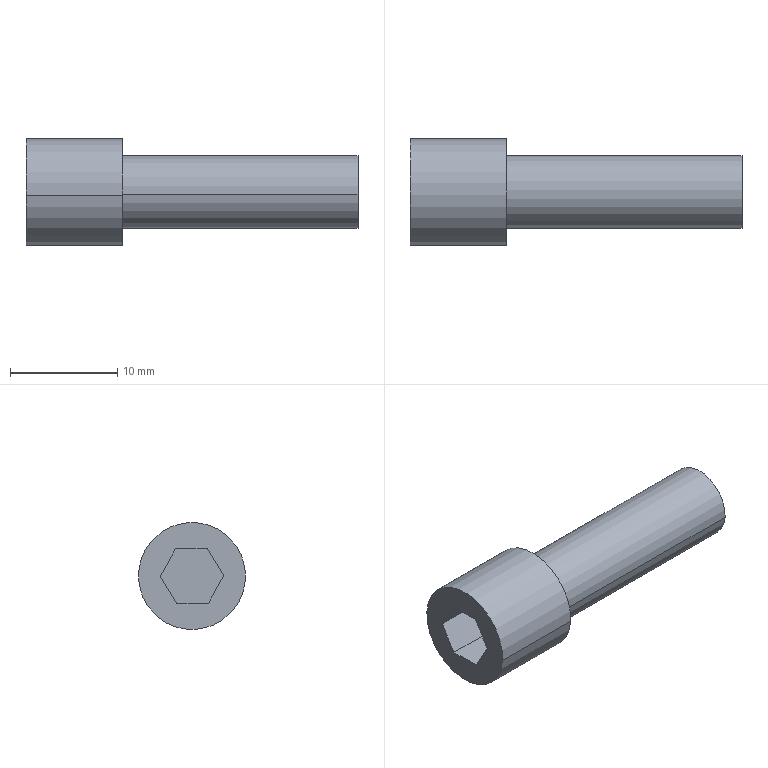Component | SolidWorks | ScrewM8X20-2 | 1 solid | 14 faces | box 31 x 10 x 10 mm | volume 1369 mm3 | plane 10 | cylinder 4 | commonest cylinder face diameters 10 x2 6.8 x2
STEP:
#1=CARTESIAN_POINT('',(-5.315,6.102,-2.114));
#2=VERTEX_POINT('',#1);
#3=CARTESIAN_POINT('',(-5.315,5.709,-2.138));
#4=VERTEX_POINT('',#3);
#5=CARTESIAN_POINT('',(-5.315,5.906,-2.126));
#6=DIRECTION('',(-1.,0.,0.));
#7=DIRECTION('',(0.,0.998,0.06334));
#8=AXIS2_PLACEMENT_3D('',#5,#6,#7);
#9=CIRCLE('',#8,0.1969);
#10=EDGE_CURVE('',#2,#4,#9,.T.);
#11=ORIENTED_EDGE('',*,*,#10,.F.);
#12=CARTESIAN_POINT('',(-4.961,6.102,-2.114));
#13=VERTEX_POINT('',#12);
#14=CARTESIAN_POINT('',(-5.315,6.102,-2.114));
#15=DIRECTION('',(1.,-0.,-0.));
#16=VECTOR('',#15,39.37);
#17=LINE('',#14,#16);
#18=EDGE_CURVE('',#2,#13,#17,.T.);
#19=ORIENTED_EDGE('',*,*,#18,.T.);
#20=CARTESIAN_POINT('',(-4.961,5.709,-2.138));
#21=VERTEX_POINT('',#20);
#22=CARTESIAN_POINT('',(-4.961,5.906,-2.126));
#23=DIRECTION('',(-1.,0.,0.));
#24=DIRECTION('',(0.,0.998,0.06334));
#25=AXIS2_PLACEMENT_3D('',#22,#23,#24);
#26=CIRCLE('',#25,0.1969);
#27=EDGE_CURVE('',#13,#21,#26,.T.);
#28=ORIENTED_EDGE('',*,*,#27,.T.);
#29=CARTESIAN_POINT('',(-5.315,5.709,-2.138));
#30=DIRECTION('',(1.,-0.,-0.));
#31=VECTOR('',#30,39.37);
#32=LINE('',#29,#31);
#33=EDGE_CURVE('',#4,#21,#32,.T.);
#34=ORIENTED_EDGE('',*,*,#33,.F.);
#35=EDGE_LOOP('',(#11,#19,#28,#34));
#36=FACE_OUTER_BOUND('',#35,.T.);
#37=CARTESIAN_POINT('',(-5.315,5.906,-2.126));
#38=DIRECTION('',(1.,-0.,-0.));
#39=DIRECTION('',(0.,-0.998,-0.06334));
#40=AXIS2_PLACEMENT_3D('',#37,#38,#39);
#41=CYLINDRICAL_SURFACE('',#40,0.1969);
#42=ADVANCED_FACE('',(#36),#41,.T.);
#43=CARTESIAN_POINT('',(-4.094,6.039,-2.118));
#44=VERTEX_POINT('',#43);
#45=CARTESIAN_POINT('',(-4.094,5.772,-2.134));
#46=VERTEX_POINT('',#45);
#47=CARTESIAN_POINT('',(-4.094,5.906,-2.126));
#48=DIRECTION('',(-1.,0.,0.));
#49=DIRECTION('',(0.,0.998,0.06334));
#50=AXIS2_PLACEMENT_3D('',#47,#48,#49);
#51=CIRCLE('',#50,0.1339);
#52=EDGE_CURVE('',#44,#46,#51,.T.);
#53=ORIENTED_EDGE('',*,*,#52,.T.);
#54=CARTESIAN_POINT('',(-4.961,5.772,-2.134));
#55=VERTEX_POINT('',#54);
#56=CARTESIAN_POINT('',(-4.094,5.772,-2.134));
#57=DIRECTION('',(-1.,0.,0.));
#58=VECTOR('',#57,39.37);
#59=LINE('',#56,#58);
#60=EDGE_CURVE('',#46,#55,#59,.T.);
#61=ORIENTED_EDGE('',*,*,#60,.T.);
#62=CARTESIAN_POINT('',(-4.961,6.039,-2.118));
#63=VERTEX_POINT('',#62);
#64=CARTESIAN_POINT('',(-4.961,5.906,-2.126));
#65=DIRECTION('',(-1.,0.,0.));
#66=DIRECTION('',(0.,0.998,0.06334));
#67=AXIS2_PLACEMENT_3D('',#64,#65,#66);
#68=CIRCLE('',#67,0.1339);
#69=EDGE_CURVE('',#63,#55,#68,.T.);
#70=ORIENTED_EDGE('',*,*,#69,.F.);
#71=CARTESIAN_POINT('',(-4.094,6.039,-2.118));
#72=DIRECTION('',(-1.,0.,0.));
#73=VECTOR('',#72,39.37);
#74=LINE('',#71,#73);
#75=EDGE_CURVE('',#44,#63,#74,.T.);
#76=ORIENTED_EDGE('',*,*,#75,.F.);
#77=EDGE_LOOP('',(#53,#61,#70,#76));
#78=FACE_OUTER_BOUND('',#77,.T.);
#79=CARTESIAN_POINT('',(-4.094,5.906,-2.126));
#80=DIRECTION('',(-1.,0.,0.));
#81=DIRECTION('',(0.,0.998,0.06334));
#82=AXIS2_PLACEMENT_3D('',#79,#80,#81);
#83=CYLINDRICAL_SURFACE('',#82,0.1339);
#84=ADVANCED_FACE('',(#78),#83,.T.);
#85=ORIENTED_EDGE('',*,*,#60,.F.);
#86=CARTESIAN_POINT('',(-4.094,5.906,-2.126));
#87=DIRECTION('',(-1.,0.,0.));
#88=DIRECTION('',(0.,0.998,0.06334));
#89=AXIS2_PLACEMENT_3D('',#86,#87,#88);
#90=CIRCLE('',#89,0.1339);
#91=EDGE_CURVE('',#46,#44,#90,.T.);
#92=ORIENTED_EDGE('',*,*,#91,.T.);
#93=ORIENTED_EDGE('',*,*,#75,.T.);
#94=CARTESIAN_POINT('',(-4.961,5.906,-2.126));
#95=DIRECTION('',(-1.,0.,0.));
#96=DIRECTION('',(0.,0.998,0.06334));
#97=AXIS2_PLACEMENT_3D('',#94,#95,#96);
#98=CIRCLE('',#97,0.1339);
#99=EDGE_CURVE('',#55,#63,#98,.T.);
#100=ORIENTED_EDGE('',*,*,#99,.F.);
#101=EDGE_LOOP('',(#85,#92,#93,#100));
#102=FACE_OUTER_BOUND('',#101,.T.);
#103=CARTESIAN_POINT('',(-4.094,5.906,-2.126));
#104=DIRECTION('',(-1.,0.,0.));
#105=DIRECTION('',(0.,0.998,0.06334));
#106=AXIS2_PLACEMENT_3D('',#103,#104,#105);
#107=CYLINDRICAL_SURFACE('',#106,0.1339);
#108=ADVANCED_FACE('',(#102),#107,.T.);
#109=ORIENTED_EDGE('',*,*,#52,.F.);
#110=ORIENTED_EDGE('',*,*,#91,.F.);
#111=EDGE_LOOP('',(#109,#110));
#112=FACE_OUTER_BOUND('',#111,.T.);
#113=CARTESIAN_POINT('',(-4.094,5.906,-2.126));
#114=DIRECTION('',(-1.,0.,0.));
#115=DIRECTION('',(0.,0.998,0.06334));
#116=AXIS2_PLACEMENT_3D('',#113,#114,#115);
#117=PLANE('',#116);
#118=ADVANCED_FACE('',(#112),#117,.F.);
#119=ORIENTED_EDGE('',*,*,#18,.F.);
#120=CARTESIAN_POINT('',(-5.315,5.906,-2.126));
#121=DIRECTION('',(-1.,0.,0.));
#122=DIRECTION('',(0.,0.998,0.06334));
#123=AXIS2_PLACEMENT_3D('',#120,#121,#122);
#124=CIRCLE('',#123,0.1969);
#125=EDGE_CURVE('',#4,#2,#124,.T.);
#126=ORIENTED_EDGE('',*,*,#125,.F.);
#127=ORIENTED_EDGE('',*,*,#33,.T.);
#128=CARTESIAN_POINT('',(-4.961,5.906,-2.126));
#129=DIRECTION('',(-1.,0.,0.));
#130=DIRECTION('',(0.,0.998,0.06334));
#131=AXIS2_PLACEMENT_3D('',#128,#129,#130);
#132=CIRCLE('',#131,0.1969);
#133=EDGE_CURVE('',#21,#13,#132,.T.);
#134=ORIENTED_EDGE('',*,*,#133,.T.);
#135=EDGE_LOOP('',(#119,#126,#127,#134));
#136=FACE_OUTER_BOUND('',#135,.T.);
#137=CARTESIAN_POINT('',(-5.315,5.906,-2.126));
#138=DIRECTION('',(1.,-0.,-0.));
#139=DIRECTION('',(0.,-0.998,-0.06334));
#140=AXIS2_PLACEMENT_3D('',#137,#138,#139);
#141=CYLINDRICAL_SURFACE('',#140,0.1969);
#142=ADVANCED_FACE('',(#136),#141,.T.);
#143=CARTESIAN_POINT('',(-5.315,6.022,-2.129));
#144=VERTEX_POINT('',#143);
#145=CARTESIAN_POINT('',(-5.315,5.962,-2.228));
#146=VERTEX_POINT('',#145);
#147=CARTESIAN_POINT('',(-5.315,6.022,-2.129));
#148=DIRECTION('',(-0.,-0.5195,-0.8544));
#149=VECTOR('',#148,39.37);
#150=LINE('',#147,#149);
#151=EDGE_CURVE('',#144,#146,#150,.T.);
#152=ORIENTED_EDGE('',*,*,#151,.F.);
#153=CARTESIAN_POINT('',(-5.315,5.966,-2.026));
#154=VERTEX_POINT('',#153);
#155=CARTESIAN_POINT('',(-5.315,5.966,-2.026));
#156=DIRECTION('',(-0.,0.4802,-0.8772));
#157=VECTOR('',#156,39.37);
#158=LINE('',#155,#157);
#159=EDGE_CURVE('',#154,#144,#158,.T.);
#160=ORIENTED_EDGE('',*,*,#159,.F.);
#161=CARTESIAN_POINT('',(-5.315,5.849,-2.024));
#162=VERTEX_POINT('',#161);
#163=CARTESIAN_POINT('',(-5.315,5.849,-2.024));
#164=DIRECTION('',(0.,0.9997,-0.02271));
#165=VECTOR('',#164,39.37);
#166=LINE('',#163,#165);
#167=EDGE_CURVE('',#162,#154,#166,.T.);
#168=ORIENTED_EDGE('',*,*,#167,.F.);
#169=CARTESIAN_POINT('',(-5.315,5.789,-2.123));
#170=VERTEX_POINT('',#169);
#171=CARTESIAN_POINT('',(-5.315,5.789,-2.123));
#172=DIRECTION('',(0.,0.5195,0.8544));
#173=VECTOR('',#172,39.37);
#174=LINE('',#171,#173);
#175=EDGE_CURVE('',#170,#162,#174,.T.);
#176=ORIENTED_EDGE('',*,*,#175,.F.);
#177=CARTESIAN_POINT('',(-5.315,5.845,-2.226));
#178=VERTEX_POINT('',#177);
#179=CARTESIAN_POINT('',(-5.315,5.845,-2.226));
#180=DIRECTION('',(0.,-0.4802,0.8772));
#181=VECTOR('',#180,39.37);
#182=LINE('',#179,#181);
#183=EDGE_CURVE('',#178,#170,#182,.T.);
#184=ORIENTED_EDGE('',*,*,#183,.F.);
#185=CARTESIAN_POINT('',(-5.315,5.962,-2.228));
#186=DIRECTION('',(-0.,-0.9997,0.02271));
#187=VECTOR('',#186,39.37);
#188=LINE('',#185,#187);
#189=EDGE_CURVE('',#146,#178,#188,.T.);
#190=ORIENTED_EDGE('',*,*,#189,.F.);
#191=EDGE_LOOP('',(#152,#160,#168,#176,#184,#190));
#192=FACE_BOUND('',#191,.T.);
#193=ORIENTED_EDGE('',*,*,#125,.T.);
#194=ORIENTED_EDGE('',*,*,#10,.T.);
#195=EDGE_LOOP('',(#193,#194));
#196=FACE_OUTER_BOUND('',#195,.T.);
#197=CARTESIAN_POINT('',(-5.315,5.906,-2.126));
#198=DIRECTION('',(-1.,0.,0.));
#199=DIRECTION('',(0.,0.998,0.06334));
#200=AXIS2_PLACEMENT_3D('',#197,#198,#199);
#201=PLANE('',#200);
#202=ADVANCED_FACE('',(#192,#196),#201,.T.);
#203=ORIENTED_EDGE('',*,*,#69,.T.);
#204=ORIENTED_EDGE('',*,*,#99,.T.);
#205=EDGE_LOOP('',(#203,#204));
#206=FACE_BOUND('',#205,.T.);
#207=ORIENTED_EDGE('',*,*,#133,.F.);
#208=ORIENTED_EDGE('',*,*,#27,.F.);
#209=EDGE_LOOP('',(#207,#208));
#210=FACE_OUTER_BOUND('',#209,.T.);
#211=CARTESIAN_POINT('',(-4.961,5.906,-2.126));
#212=DIRECTION('',(-1.,0.,0.));
#213=DIRECTION('',(0.,0.998,0.06334));
#214=AXIS2_PLACEMENT_3D('',#211,#212,#213);
#215=PLANE('',#214);
#216=ADVANCED_FACE('',(#206,#210),#215,.F.);
#217=ORIENTED_EDGE('',*,*,#151,.T.);
#218=CARTESIAN_POINT('',(-5.079,5.962,-2.228));
#219=VERTEX_POINT('',#218);
#220=CARTESIAN_POINT('',(-5.079,5.962,-2.228));
#221=DIRECTION('',(-1.,0.,0.));
#222=VECTOR('',#221,39.37);
#223=LINE('',#220,#222);
#224=EDGE_CURVE('',#219,#146,#223,.T.);
#225=ORIENTED_EDGE('',*,*,#224,.F.);
#226=CARTESIAN_POINT('',(-5.079,6.022,-2.129));
#227=VERTEX_POINT('',#226);
#228=CARTESIAN_POINT('',(-5.079,6.022,-2.129));
#229=DIRECTION('',(-0.,-0.5195,-0.8544));
#230=VECTOR('',#229,39.37);
#231=LINE('',#228,#230);
#232=EDGE_CURVE('',#227,#219,#231,.T.);
#233=ORIENTED_EDGE('',*,*,#232,.F.);
#234=CARTESIAN_POINT('',(-5.079,6.022,-2.129));
#235=DIRECTION('',(-1.,0.,0.));
#236=VECTOR('',#235,39.37);
#237=LINE('',#234,#236);
#238=EDGE_CURVE('',#227,#144,#237,.T.);
#239=ORIENTED_EDGE('',*,*,#238,.T.);
#240=EDGE_LOOP('',(#217,#225,#233,#239));
#241=FACE_OUTER_BOUND('',#240,.T.);
#242=CARTESIAN_POINT('',(-5.079,6.022,-2.129));
#243=DIRECTION('',(0.,0.8544,-0.5195));
#244=DIRECTION('',(-0.,-0.5195,-0.8544));
#245=AXIS2_PLACEMENT_3D('',#242,#243,#244);
#246=PLANE('',#245);
#247=ADVANCED_FACE('',(#241),#246,.F.);
#248=ORIENTED_EDGE('',*,*,#159,.T.);
#249=ORIENTED_EDGE('',*,*,#238,.F.);
#250=CARTESIAN_POINT('',(-5.079,5.966,-2.026));
#251=VERTEX_POINT('',#250);
#252=CARTESIAN_POINT('',(-5.079,5.966,-2.026));
#253=DIRECTION('',(-0.,0.4802,-0.8772));
#254=VECTOR('',#253,39.37);
#255=LINE('',#252,#254);
#256=EDGE_CURVE('',#251,#227,#255,.T.);
#257=ORIENTED_EDGE('',*,*,#256,.F.);
#258=CARTESIAN_POINT('',(-5.079,5.966,-2.026));
#259=DIRECTION('',(-1.,0.,0.));
#260=VECTOR('',#259,39.37);
#261=LINE('',#258,#260);
#262=EDGE_CURVE('',#251,#154,#261,.T.);
#263=ORIENTED_EDGE('',*,*,#262,.T.);
#264=EDGE_LOOP('',(#248,#249,#257,#263));
#265=FACE_OUTER_BOUND('',#264,.T.);
#266=CARTESIAN_POINT('',(-5.079,5.966,-2.026));
#267=DIRECTION('',(0.,0.8772,0.4802));
#268=DIRECTION('',(-0.,0.4802,-0.8772));
#269=AXIS2_PLACEMENT_3D('',#266,#267,#268);
#270=PLANE('',#269);
#271=ADVANCED_FACE('',(#265),#270,.F.);
#272=ORIENTED_EDGE('',*,*,#167,.T.);
#273=ORIENTED_EDGE('',*,*,#262,.F.);
#274=CARTESIAN_POINT('',(-5.079,5.849,-2.024));
#275=VERTEX_POINT('',#274);
#276=CARTESIAN_POINT('',(-5.079,5.849,-2.024));
#277=DIRECTION('',(0.,0.9997,-0.02271));
#278=VECTOR('',#277,39.37);
#279=LINE('',#276,#278);
#280=EDGE_CURVE('',#275,#251,#279,.T.);
#281=ORIENTED_EDGE('',*,*,#280,.F.);
#282=CARTESIAN_POINT('',(-5.079,5.849,-2.024));
#283=DIRECTION('',(-1.,0.,0.));
#284=VECTOR('',#283,39.37);
#285=LINE('',#282,#284);
#286=EDGE_CURVE('',#275,#162,#285,.T.);
#287=ORIENTED_EDGE('',*,*,#286,.T.);
#288=EDGE_LOOP('',(#272,#273,#281,#287));
#289=FACE_OUTER_BOUND('',#288,.T.);
#290=CARTESIAN_POINT('',(-5.079,5.849,-2.024));
#291=DIRECTION('',(0.,0.02271,0.9997));
#292=DIRECTION('',(0.,0.9997,-0.02271));
#293=AXIS2_PLACEMENT_3D('',#290,#291,#292);
#294=PLANE('',#293);
#295=ADVANCED_FACE('',(#289),#294,.F.);
#296=ORIENTED_EDGE('',*,*,#175,.T.);
#297=ORIENTED_EDGE('',*,*,#286,.F.);
#298=CARTESIAN_POINT('',(-5.079,5.789,-2.123));
#299=VERTEX_POINT('',#298);
#300=CARTESIAN_POINT('',(-5.079,5.789,-2.123));
#301=DIRECTION('',(0.,0.5195,0.8544));
#302=VECTOR('',#301,39.37);
#303=LINE('',#300,#302);
#304=EDGE_CURVE('',#299,#275,#303,.T.);
#305=ORIENTED_EDGE('',*,*,#304,.F.);
#306=CARTESIAN_POINT('',(-5.079,5.789,-2.123));
#307=DIRECTION('',(-1.,0.,0.));
#308=VECTOR('',#307,39.37);
#309=LINE('',#306,#308);
#310=EDGE_CURVE('',#299,#170,#309,.T.);
#311=ORIENTED_EDGE('',*,*,#310,.T.);
#312=EDGE_LOOP('',(#296,#297,#305,#311));
#313=FACE_OUTER_BOUND('',#312,.T.);
#314=CARTESIAN_POINT('',(-5.079,5.789,-2.123));
#315=DIRECTION('',(-0.,-0.8544,0.5195));
#316=DIRECTION('',(0.,0.5195,0.8544));
#317=AXIS2_PLACEMENT_3D('',#314,#315,#316);
#318=PLANE('',#317);
#319=ADVANCED_FACE('',(#313),#318,.F.);
#320=ORIENTED_EDGE('',*,*,#183,.T.);
#321=ORIENTED_EDGE('',*,*,#310,.F.);
#322=CARTESIAN_POINT('',(-5.079,5.845,-2.226));
#323=VERTEX_POINT('',#322);
#324=CARTESIAN_POINT('',(-5.079,5.845,-2.226));
#325=DIRECTION('',(0.,-0.4802,0.8772));
#326=VECTOR('',#325,39.37);
#327=LINE('',#324,#326);
#328=EDGE_CURVE('',#323,#299,#327,.T.);
#329=ORIENTED_EDGE('',*,*,#328,.F.);
#330=CARTESIAN_POINT('',(-5.079,5.845,-2.226));
#331=DIRECTION('',(-1.,0.,0.));
#332=VECTOR('',#331,39.37);
#333=LINE('',#330,#332);
#334=EDGE_CURVE('',#323,#178,#333,.T.);
#335=ORIENTED_EDGE('',*,*,#334,.T.);
#336=EDGE_LOOP('',(#320,#321,#329,#335));
#337=FACE_OUTER_BOUND('',#336,.T.);
#338=CARTESIAN_POINT('',(-5.079,5.845,-2.226));
#339=DIRECTION('',(-0.,-0.8772,-0.4802));
#340=DIRECTION('',(0.,-0.4802,0.8772));
#341=AXIS2_PLACEMENT_3D('',#338,#339,#340);
#342=PLANE('',#341);
#343=ADVANCED_FACE('',(#337),#342,.F.);
#344=ORIENTED_EDGE('',*,*,#189,.T.);
#345=ORIENTED_EDGE('',*,*,#334,.F.);
#346=CARTESIAN_POINT('',(-5.079,5.962,-2.228));
#347=DIRECTION('',(-0.,-0.9997,0.02271));
#348=VECTOR('',#347,39.37);
#349=LINE('',#346,#348);
#350=EDGE_CURVE('',#219,#323,#349,.T.);
#351=ORIENTED_EDGE('',*,*,#350,.F.);
#352=ORIENTED_EDGE('',*,*,#224,.T.);
#353=EDGE_LOOP('',(#344,#345,#351,#352));
#354=FACE_OUTER_BOUND('',#353,.T.);
#355=CARTESIAN_POINT('',(-5.079,5.962,-2.228));
#356=DIRECTION('',(-0.,-0.02271,-0.9997));
#357=DIRECTION('',(-0.,-0.9997,0.02271));
#358=AXIS2_PLACEMENT_3D('',#355,#356,#357);
#359=PLANE('',#358);
#360=ADVANCED_FACE('',(#354),#359,.F.);
#361=ORIENTED_EDGE('',*,*,#232,.T.);
#362=ORIENTED_EDGE('',*,*,#350,.T.);
#363=ORIENTED_EDGE('',*,*,#328,.T.);
#364=ORIENTED_EDGE('',*,*,#304,.T.);
#365=ORIENTED_EDGE('',*,*,#280,.T.);
#366=ORIENTED_EDGE('',*,*,#256,.T.);
#367=EDGE_LOOP('',(#361,#362,#363,#364,#365,#366));
#368=FACE_OUTER_BOUND('',#367,.T.);
#369=CARTESIAN_POINT('',(-5.079,6.024,5.337));
#370=DIRECTION('',(-1.,0.,0.));
#371=DIRECTION('',(0.,0.998,0.06334));
#372=AXIS2_PLACEMENT_3D('',#369,#370,#371);
#373=PLANE('',#372);
#374=ADVANCED_FACE('',(#368),#373,.T.);
#375=CLOSED_SHELL('',(#42,#84,#108,#118,#142,#202,#216,#247,#271,#295,#319,#343,#360,#374));
#376=MANIFOLD_SOLID_BREP('',#375);
#377=CARTESIAN_POINT('',(0.,0.,0.));
#378=DIRECTION('',(0.,0.,1.));
#379=DIRECTION('',(1.,0.,0.));
#380=AXIS2_PLACEMENT_3D('',#377,#378,#379);
#381=(LENGTH_UNIT()NAMED_UNIT(*)SI_UNIT($,.METRE.));
#382=LENGTH_MEASURE_WITH_UNIT(LENGTH_MEASURE(0.0254),#381);
#383=DIMENSIONAL_EXPONENTS(1.,0.,0.,0.,0.,0.,0.);
#384=(CONVERSION_BASED_UNIT('',#382)LENGTH_UNIT()NAMED_UNIT(#383));
#385=UNCERTAINTY_MEASURE_WITH_UNIT(LENGTH_MEASURE(0.00001),#384,'','');
#386=(NAMED_UNIT(*)PLANE_ANGLE_UNIT()SI_UNIT($,.RADIAN.));
#387=(NAMED_UNIT(*)SI_UNIT($,.STERADIAN.)SOLID_ANGLE_UNIT());
#388=(GEOMETRIC_REPRESENTATION_CONTEXT(3)GLOBAL_UNCERTAINTY_ASSIGNED_CONTEXT((#385))GLOBAL_UNIT_ASSIGNED_CONTEXT((#384,#386,#387))REPRESENTATION_CONTEXT('',''));
#389=ADVANCED_BREP_SHAPE_REPRESENTATION('',(#376,#380),#388);
#390=COLOUR_RGB('',0.7922,0.8196,0.9333);
#391=FILL_AREA_STYLE_COLOUR('',#390);
#392=FILL_AREA_STYLE('',(#391));
#393=SURFACE_STYLE_FILL_AREA(#392);
#394=SURFACE_SIDE_STYLE('',(#393));
#395=SURFACE_STYLE_USAGE(.BOTH.,#394);
#396=PRESENTATION_STYLE_ASSIGNMENT((#395));
#397=STYLED_ITEM('',(#396),#376);
#398=(LENGTH_UNIT()NAMED_UNIT(*)SI_UNIT($,.METRE.));
#399=LENGTH_MEASURE_WITH_UNIT(LENGTH_MEASURE(0.0254),#398);
#400=DIMENSIONAL_EXPONENTS(1.,0.,0.,0.,0.,0.,0.);
#401=(CONVERSION_BASED_UNIT('',#399)LENGTH_UNIT()NAMED_UNIT(#400));
#402=UNCERTAINTY_MEASURE_WITH_UNIT(LENGTH_MEASURE(0.00001),#401,'','');
#403=(NAMED_UNIT(*)PLANE_ANGLE_UNIT()SI_UNIT($,.RADIAN.));
#404=(NAMED_UNIT(*)SI_UNIT($,.STERADIAN.)SOLID_ANGLE_UNIT());
#405=(GEOMETRIC_REPRESENTATION_CONTEXT(3)GLOBAL_UNCERTAINTY_ASSIGNED_CONTEXT((#402))GLOBAL_UNIT_ASSIGNED_CONTEXT((#401,#403,#404))REPRESENTATION_CONTEXT('',''));
#406=MECHANICAL_DESIGN_GEOMETRIC_PRESENTATION_REPRESENTATION('',(#397),#405);
#407=PRESENTATION_LAYER_ASSIGNMENT('','',(#397));